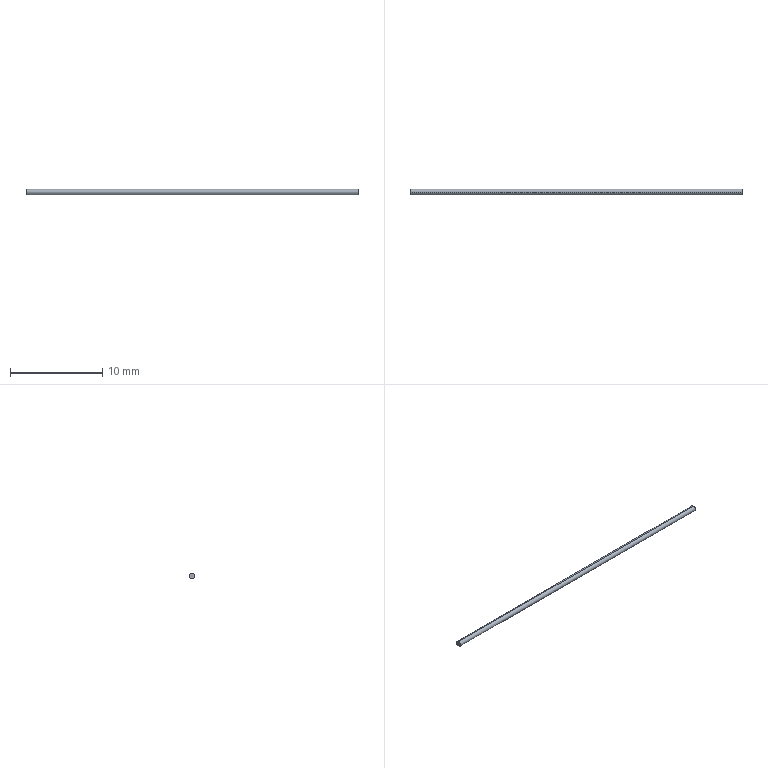Component | SolidWorks | PurchasedPart_ResistanceWireL50-1 | 1 solid | 4 faces | box 36 x 0.6 x 0.6 mm | volume 10 mm3 | cylinder 2 | plane 2 | commonest cylinder face diameters 0.6 x2
build123d program:
from build123d import *

# Parameters (mm, degrees)
SKETCH1_R           = 0.3
BOSS_EXTRUDE1_DEPTH = 36


with BuildPart() as part:
    # Sketch1 → Boss-Extrude1 (new body)
    with BuildSketch(Plane.XY):
        Circle(SKETCH1_R)
    extrude(amount=BOSS_EXTRUDE1_DEPTH)


solid = part.part

# Placed as in the assembly
solid = solid.moved(Location((81.712, -108.5, 217), (0, 90, 0)))
STEP:
#1=CARTESIAN_POINT('',(3.217,-4.272,8.555));
#2=VERTEX_POINT('',#1);
#3=CARTESIAN_POINT('',(3.217,-4.271,8.532));
#4=VERTEX_POINT('',#3);
#5=CARTESIAN_POINT('',(3.217,-4.272,8.543));
#6=DIRECTION('',(-1.,-0.,-0.));
#7=DIRECTION('',(0.,-0.0324,0.9995));
#8=AXIS2_PLACEMENT_3D('',#5,#6,#7);
#9=CIRCLE('',#8,0.01181);
#10=EDGE_CURVE('',#2,#4,#9,.T.);
#11=ORIENTED_EDGE('',*,*,#10,.F.);
#12=CARTESIAN_POINT('',(4.634,-4.272,8.555));
#13=VERTEX_POINT('',#12);
#14=CARTESIAN_POINT('',(3.217,-4.272,8.555));
#15=DIRECTION('',(1.,0.,0.));
#16=VECTOR('',#15,39.37);
#17=LINE('',#14,#16);
#18=EDGE_CURVE('',#2,#13,#17,.T.);
#19=ORIENTED_EDGE('',*,*,#18,.T.);
#20=CARTESIAN_POINT('',(4.634,-4.271,8.532));
#21=VERTEX_POINT('',#20);
#22=CARTESIAN_POINT('',(4.634,-4.272,8.543));
#23=DIRECTION('',(-1.,-0.,-0.));
#24=DIRECTION('',(0.,-0.0324,0.9995));
#25=AXIS2_PLACEMENT_3D('',#22,#23,#24);
#26=CIRCLE('',#25,0.01181);
#27=EDGE_CURVE('',#13,#21,#26,.T.);
#28=ORIENTED_EDGE('',*,*,#27,.T.);
#29=CARTESIAN_POINT('',(3.217,-4.271,8.532));
#30=DIRECTION('',(1.,0.,0.));
#31=VECTOR('',#30,39.37);
#32=LINE('',#29,#31);
#33=EDGE_CURVE('',#4,#21,#32,.T.);
#34=ORIENTED_EDGE('',*,*,#33,.F.);
#35=EDGE_LOOP('',(#11,#19,#28,#34));
#36=FACE_OUTER_BOUND('',#35,.T.);
#37=CARTESIAN_POINT('',(3.217,-4.272,8.543));
#38=DIRECTION('',(1.,0.,0.));
#39=DIRECTION('',(0.,0.0324,-0.9995));
#40=AXIS2_PLACEMENT_3D('',#37,#38,#39);
#41=CYLINDRICAL_SURFACE('',#40,0.01181);
#42=ADVANCED_FACE('',(#36),#41,.T.);
#43=ORIENTED_EDGE('',*,*,#18,.F.);
#44=CARTESIAN_POINT('',(3.217,-4.272,8.543));
#45=DIRECTION('',(-1.,-0.,-0.));
#46=DIRECTION('',(0.,-0.0324,0.9995));
#47=AXIS2_PLACEMENT_3D('',#44,#45,#46);
#48=CIRCLE('',#47,0.01181);
#49=EDGE_CURVE('',#4,#2,#48,.T.);
#50=ORIENTED_EDGE('',*,*,#49,.F.);
#51=ORIENTED_EDGE('',*,*,#33,.T.);
#52=CARTESIAN_POINT('',(4.634,-4.272,8.543));
#53=DIRECTION('',(-1.,-0.,-0.));
#54=DIRECTION('',(0.,-0.0324,0.9995));
#55=AXIS2_PLACEMENT_3D('',#52,#53,#54);
#56=CIRCLE('',#55,0.01181);
#57=EDGE_CURVE('',#21,#13,#56,.T.);
#58=ORIENTED_EDGE('',*,*,#57,.T.);
#59=EDGE_LOOP('',(#43,#50,#51,#58));
#60=FACE_OUTER_BOUND('',#59,.T.);
#61=CARTESIAN_POINT('',(3.217,-4.272,8.543));
#62=DIRECTION('',(1.,0.,0.));
#63=DIRECTION('',(0.,0.0324,-0.9995));
#64=AXIS2_PLACEMENT_3D('',#61,#62,#63);
#65=CYLINDRICAL_SURFACE('',#64,0.01181);
#66=ADVANCED_FACE('',(#60),#65,.T.);
#67=ORIENTED_EDGE('',*,*,#49,.T.);
#68=ORIENTED_EDGE('',*,*,#10,.T.);
#69=EDGE_LOOP('',(#67,#68));
#70=FACE_OUTER_BOUND('',#69,.T.);
#71=CARTESIAN_POINT('',(3.217,-4.272,8.543));
#72=DIRECTION('',(-1.,-0.,-0.));
#73=DIRECTION('',(-0.,-0.0324,0.9995));
#74=AXIS2_PLACEMENT_3D('',#71,#72,#73);
#75=PLANE('',#74);
#76=ADVANCED_FACE('',(#70),#75,.T.);
#77=ORIENTED_EDGE('',*,*,#57,.F.);
#78=ORIENTED_EDGE('',*,*,#27,.F.);
#79=EDGE_LOOP('',(#77,#78));
#80=FACE_OUTER_BOUND('',#79,.T.);
#81=CARTESIAN_POINT('',(4.634,-4.272,8.543));
#82=DIRECTION('',(-1.,-0.,-0.));
#83=DIRECTION('',(-0.,-0.0324,0.9995));
#84=AXIS2_PLACEMENT_3D('',#81,#82,#83);
#85=PLANE('',#84);
#86=ADVANCED_FACE('',(#80),#85,.F.);
#87=CLOSED_SHELL('',(#42,#66,#76,#86));
#88=MANIFOLD_SOLID_BREP('',#87);
#89=CARTESIAN_POINT('',(0.,0.,0.));
#90=DIRECTION('',(0.,0.,1.));
#91=DIRECTION('',(1.,0.,0.));
#92=AXIS2_PLACEMENT_3D('',#89,#90,#91);
#93=(LENGTH_UNIT()NAMED_UNIT(*)SI_UNIT($,.METRE.));
#94=LENGTH_MEASURE_WITH_UNIT(LENGTH_MEASURE(0.0254),#93);
#95=DIMENSIONAL_EXPONENTS(1.,0.,0.,0.,0.,0.,0.);
#96=(CONVERSION_BASED_UNIT('',#94)LENGTH_UNIT()NAMED_UNIT(#95));
#97=UNCERTAINTY_MEASURE_WITH_UNIT(LENGTH_MEASURE(0.00001),#96,'','');
#98=(NAMED_UNIT(*)PLANE_ANGLE_UNIT()SI_UNIT($,.RADIAN.));
#99=(NAMED_UNIT(*)SI_UNIT($,.STERADIAN.)SOLID_ANGLE_UNIT());
#100=(GEOMETRIC_REPRESENTATION_CONTEXT(3)GLOBAL_UNCERTAINTY_ASSIGNED_CONTEXT((#97))GLOBAL_UNIT_ASSIGNED_CONTEXT((#96,#98,#99))REPRESENTATION_CONTEXT('',''));
#101=ADVANCED_BREP_SHAPE_REPRESENTATION('',(#88,#92),#100);
#102=COLOUR_RGB('',0.7922,0.8196,0.9333);
#103=FILL_AREA_STYLE_COLOUR('',#102);
#104=FILL_AREA_STYLE('',(#103));
#105=SURFACE_STYLE_FILL_AREA(#104);
#106=SURFACE_SIDE_STYLE('',(#105));
#107=SURFACE_STYLE_USAGE(.BOTH.,#106);
#108=PRESENTATION_STYLE_ASSIGNMENT((#107));
#109=STYLED_ITEM('',(#108),#88);
#110=PRESENTATION_LAYER_ASSIGNMENT('','',(#109));
#111=(LENGTH_UNIT()NAMED_UNIT(*)SI_UNIT($,.METRE.));
#112=LENGTH_MEASURE_WITH_UNIT(LENGTH_MEASURE(0.0254),#111);
#113=DIMENSIONAL_EXPONENTS(1.,0.,0.,0.,0.,0.,0.);
#114=(CONVERSION_BASED_UNIT('',#112)LENGTH_UNIT()NAMED_UNIT(#113));
#115=UNCERTAINTY_MEASURE_WITH_UNIT(LENGTH_MEASURE(0.00001),#114,'','');
#116=(NAMED_UNIT(*)PLANE_ANGLE_UNIT()SI_UNIT($,.RADIAN.));
#117=(NAMED_UNIT(*)SI_UNIT($,.STERADIAN.)SOLID_ANGLE_UNIT());
#118=(GEOMETRIC_REPRESENTATION_CONTEXT(3)GLOBAL_UNCERTAINTY_ASSIGNED_CONTEXT((#115))GLOBAL_UNIT_ASSIGNED_CONTEXT((#114,#116,#117))REPRESENTATION_CONTEXT('',''));
#119=MECHANICAL_DESIGN_GEOMETRIC_PRESENTATION_REPRESENTATION('',(#109),#118);